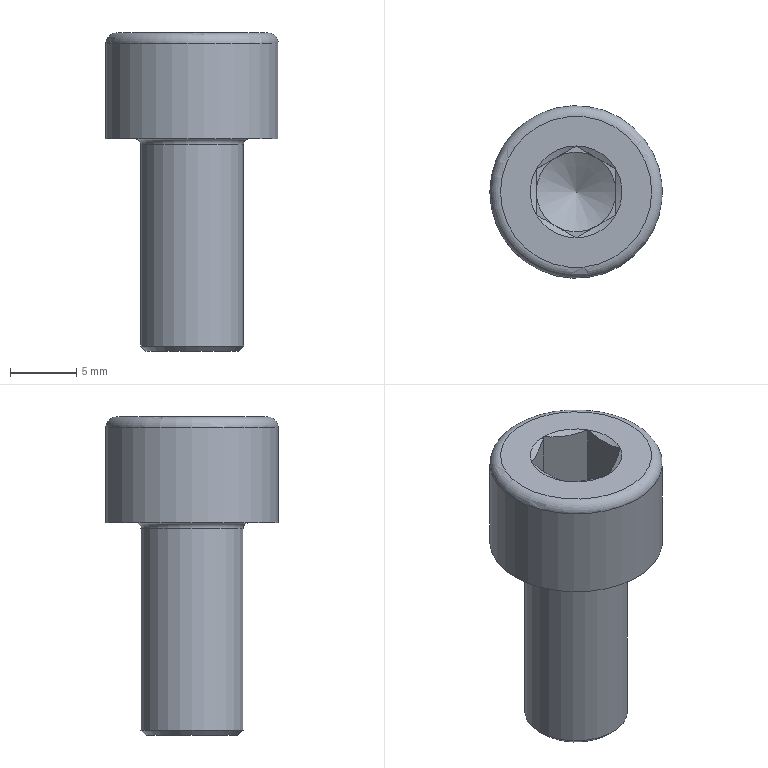Component | NX | GB-T70_1-2000_M8X16 | 1 solid | 27 faces | volume 1648 mm3 | plane 15 | cone 8 | cylinder 2 | torus 2 | commonest cylinder face diameters 7.76 x1 13 x1